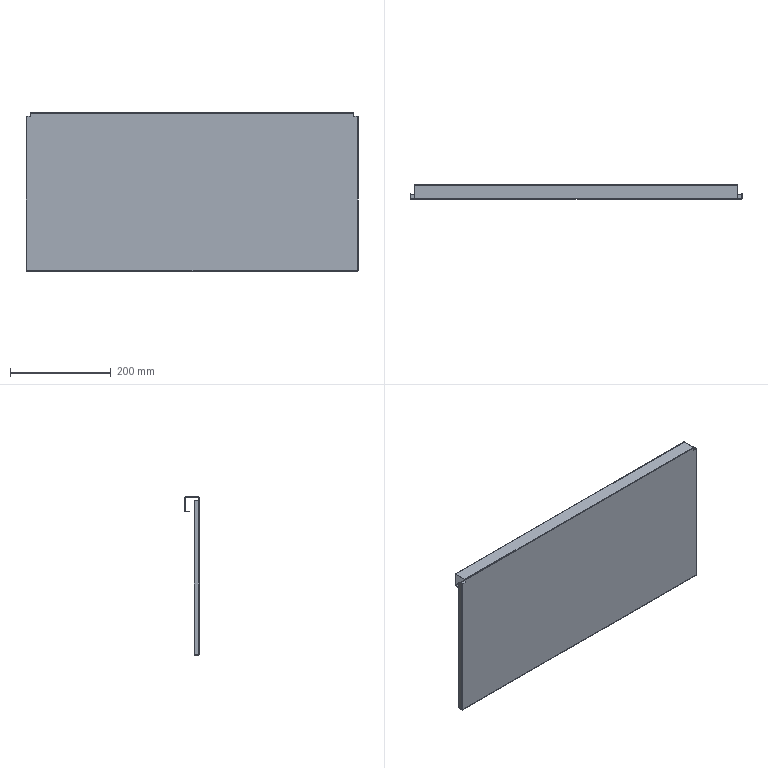Component | SolidWorks | PC-CAJ-P09-1_PM-CAJ-P39-1 | 1 solid | 58 faces | volume 179964 mm3 | plane 46 | cylinder 12 | commonest cylinder face diameters 2.4 x6 1 x6 | material Plain Carbon Steel